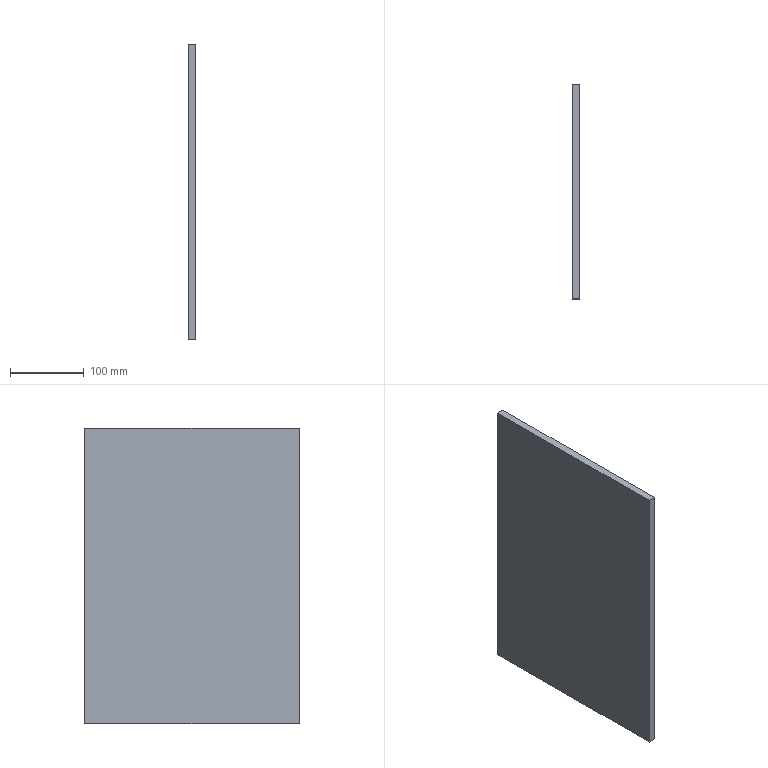Component | SolidWorks | BlockingPlate-5 | 1 solid | 6 faces | box 10 x 290 x 400 mm | volume 1160000 mm3 | plane 6 | material Plain Carbon Steel
STEP:
#1=COLOUR_RGB('',0.7922,0.8196,0.9333);
#2=FILL_AREA_STYLE_COLOUR('',#1);
#3=FILL_AREA_STYLE('',(#2));
#4=SURFACE_STYLE_FILL_AREA(#3);
#5=SURFACE_SIDE_STYLE('',(#4));
#6=SURFACE_STYLE_USAGE(.BOTH.,#5);
#7=PRESENTATION_STYLE_ASSIGNMENT((#6));
#8=CARTESIAN_POINT('',(671.454,114.953,65.169));
#9=VERTEX_POINT('',#8);
#10=CARTESIAN_POINT('',(671.454,126.37,65.169));
#11=VERTEX_POINT('',#10);
#12=CARTESIAN_POINT('',(671.454,126.37,65.169));
#13=DIRECTION('',(0.,1.,0.));
#14=VECTOR('',#13,39.37);
#15=LINE('',#12,#14);
#16=EDGE_CURVE('',#9,#11,#15,.T.);
#17=ORIENTED_EDGE('',*,*,#16,.F.);
#18=CARTESIAN_POINT('',(671.061,114.953,65.169));
#19=VERTEX_POINT('',#18);
#20=CARTESIAN_POINT('',(671.061,114.953,65.169));
#21=DIRECTION('',(1.,-0.,-0.));
#22=VECTOR('',#21,39.37);
#23=LINE('',#20,#22);
#24=EDGE_CURVE('',#19,#9,#23,.T.);
#25=ORIENTED_EDGE('',*,*,#24,.F.);
#26=CARTESIAN_POINT('',(671.061,126.37,65.169));
#27=VERTEX_POINT('',#26);
#28=CARTESIAN_POINT('',(671.061,126.37,65.169));
#29=DIRECTION('',(0.,1.,0.));
#30=VECTOR('',#29,39.37);
#31=LINE('',#28,#30);
#32=EDGE_CURVE('',#19,#27,#31,.T.);
#33=ORIENTED_EDGE('',*,*,#32,.T.);
#34=CARTESIAN_POINT('',(671.061,126.37,65.169));
#35=DIRECTION('',(1.,-0.,-0.));
#36=VECTOR('',#35,39.37);
#37=LINE('',#34,#36);
#38=EDGE_CURVE('',#27,#11,#37,.T.);
#39=ORIENTED_EDGE('',*,*,#38,.T.);
#40=EDGE_LOOP('',(#17,#25,#33,#39));
#41=FACE_OUTER_BOUND('',#40,.T.);
#42=CARTESIAN_POINT('',(671.061,126.37,65.169));
#43=DIRECTION('',(-0.,0.,-1.));
#44=DIRECTION('',(0.,1.,0.));
#45=AXIS2_PLACEMENT_3D('',#42,#43,#44);
#46=PLANE('',#45);
#47=ADVANCED_FACE('',(#41),#46,.T.);
#48=CARTESIAN_POINT('',(671.454,114.953,80.917));
#49=VERTEX_POINT('',#48);
#50=CARTESIAN_POINT('',(671.454,114.953,80.917));
#51=DIRECTION('',(-0.,0.,-1.));
#52=VECTOR('',#51,39.37);
#53=LINE('',#50,#52);
#54=EDGE_CURVE('',#49,#9,#53,.T.);
#55=ORIENTED_EDGE('',*,*,#54,.F.);
#56=CARTESIAN_POINT('',(671.061,114.953,80.917));
#57=VERTEX_POINT('',#56);
#58=CARTESIAN_POINT('',(671.061,114.953,80.917));
#59=DIRECTION('',(1.,-0.,-0.));
#60=VECTOR('',#59,39.37);
#61=LINE('',#58,#60);
#62=EDGE_CURVE('',#57,#49,#61,.T.);
#63=ORIENTED_EDGE('',*,*,#62,.F.);
#64=CARTESIAN_POINT('',(671.061,114.953,80.917));
#65=DIRECTION('',(-0.,0.,-1.));
#66=VECTOR('',#65,39.37);
#67=LINE('',#64,#66);
#68=EDGE_CURVE('',#57,#19,#67,.T.);
#69=ORIENTED_EDGE('',*,*,#68,.T.);
#70=ORIENTED_EDGE('',*,*,#24,.T.);
#71=EDGE_LOOP('',(#55,#63,#69,#70));
#72=FACE_OUTER_BOUND('',#71,.T.);
#73=CARTESIAN_POINT('',(671.061,114.953,80.917));
#74=DIRECTION('',(-0.,-1.,0.));
#75=DIRECTION('',(-0.,0.,-1.));
#76=AXIS2_PLACEMENT_3D('',#73,#74,#75);
#77=PLANE('',#76);
#78=ADVANCED_FACE('',(#72),#77,.T.);
#79=CARTESIAN_POINT('',(671.454,126.37,80.917));
#80=VERTEX_POINT('',#79);
#81=CARTESIAN_POINT('',(671.454,126.37,80.917));
#82=DIRECTION('',(-0.,-1.,-0.));
#83=VECTOR('',#82,39.37);
#84=LINE('',#81,#83);
#85=EDGE_CURVE('',#80,#49,#84,.T.);
#86=ORIENTED_EDGE('',*,*,#85,.F.);
#87=CARTESIAN_POINT('',(671.061,126.37,80.917));
#88=VERTEX_POINT('',#87);
#89=CARTESIAN_POINT('',(671.061,126.37,80.917));
#90=DIRECTION('',(1.,-0.,-0.));
#91=VECTOR('',#90,39.37);
#92=LINE('',#89,#91);
#93=EDGE_CURVE('',#88,#80,#92,.T.);
#94=ORIENTED_EDGE('',*,*,#93,.F.);
#95=CARTESIAN_POINT('',(671.061,126.37,80.917));
#96=DIRECTION('',(-0.,-1.,-0.));
#97=VECTOR('',#96,39.37);
#98=LINE('',#95,#97);
#99=EDGE_CURVE('',#88,#57,#98,.T.);
#100=ORIENTED_EDGE('',*,*,#99,.T.);
#101=ORIENTED_EDGE('',*,*,#62,.T.);
#102=EDGE_LOOP('',(#86,#94,#100,#101));
#103=FACE_OUTER_BOUND('',#102,.T.);
#104=CARTESIAN_POINT('',(671.061,126.37,80.917));
#105=DIRECTION('',(0.,-0.,1.));
#106=DIRECTION('',(-0.,-1.,-0.));
#107=AXIS2_PLACEMENT_3D('',#104,#105,#106);
#108=PLANE('',#107);
#109=ADVANCED_FACE('',(#103),#108,.T.);
#110=CARTESIAN_POINT('',(671.454,126.37,80.917));
#111=DIRECTION('',(0.,0.,1.));
#112=VECTOR('',#111,39.37);
#113=LINE('',#110,#112);
#114=EDGE_CURVE('',#11,#80,#113,.T.);
#115=ORIENTED_EDGE('',*,*,#114,.F.);
#116=ORIENTED_EDGE('',*,*,#38,.F.);
#117=CARTESIAN_POINT('',(671.061,126.37,80.917));
#118=DIRECTION('',(0.,0.,1.));
#119=VECTOR('',#118,39.37);
#120=LINE('',#117,#119);
#121=EDGE_CURVE('',#27,#88,#120,.T.);
#122=ORIENTED_EDGE('',*,*,#121,.T.);
#123=ORIENTED_EDGE('',*,*,#93,.T.);
#124=EDGE_LOOP('',(#115,#116,#122,#123));
#125=FACE_OUTER_BOUND('',#124,.T.);
#126=CARTESIAN_POINT('',(671.061,126.37,80.917));
#127=DIRECTION('',(0.,1.,-0.));
#128=DIRECTION('',(0.,0.,1.));
#129=AXIS2_PLACEMENT_3D('',#126,#127,#128);
#130=PLANE('',#129);
#131=ADVANCED_FACE('',(#125),#130,.T.);
#132=ORIENTED_EDGE('',*,*,#32,.F.);
#133=ORIENTED_EDGE('',*,*,#68,.F.);
#134=ORIENTED_EDGE('',*,*,#99,.F.);
#135=ORIENTED_EDGE('',*,*,#121,.F.);
#136=EDGE_LOOP('',(#132,#133,#134,#135));
#137=FACE_OUTER_BOUND('',#136,.T.);
#138=CARTESIAN_POINT('',(671.061,120.662,73.043));
#139=DIRECTION('',(1.,-0.,-0.));
#140=DIRECTION('',(-0.,-1.,0.));
#141=AXIS2_PLACEMENT_3D('',#138,#139,#140);
#142=PLANE('',#141);
#143=ADVANCED_FACE('',(#137),#142,.F.);
#144=ORIENTED_EDGE('',*,*,#16,.T.);
#145=ORIENTED_EDGE('',*,*,#114,.T.);
#146=ORIENTED_EDGE('',*,*,#85,.T.);
#147=ORIENTED_EDGE('',*,*,#54,.T.);
#148=EDGE_LOOP('',(#144,#145,#146,#147));
#149=FACE_OUTER_BOUND('',#148,.T.);
#150=CARTESIAN_POINT('',(671.454,120.662,73.043));
#151=DIRECTION('',(1.,-0.,-0.));
#152=DIRECTION('',(-0.,-1.,0.));
#153=AXIS2_PLACEMENT_3D('',#150,#151,#152);
#154=PLANE('',#153);
#155=ADVANCED_FACE('',(#149),#154,.T.);
#156=CLOSED_SHELL('',(#47,#78,#109,#131,#143,#155));
#157=MANIFOLD_SOLID_BREP('',#156);
#158=STYLED_ITEM('',(#7),#157);
#159=(LENGTH_UNIT()NAMED_UNIT(*)SI_UNIT($,.METRE.));
#160=LENGTH_MEASURE_WITH_UNIT(LENGTH_MEASURE(0.0254),#159);
#161=DIMENSIONAL_EXPONENTS(1.,0.,0.,0.,0.,0.,0.);
#162=(CONVERSION_BASED_UNIT('',#160)LENGTH_UNIT()NAMED_UNIT(#161));
#163=UNCERTAINTY_MEASURE_WITH_UNIT(LENGTH_MEASURE(0.00001),#162,'','');
#164=(NAMED_UNIT(*)PLANE_ANGLE_UNIT()SI_UNIT($,.RADIAN.));
#165=(NAMED_UNIT(*)SI_UNIT($,.STERADIAN.)SOLID_ANGLE_UNIT());
#166=(GEOMETRIC_REPRESENTATION_CONTEXT(3)GLOBAL_UNCERTAINTY_ASSIGNED_CONTEXT((#163))GLOBAL_UNIT_ASSIGNED_CONTEXT((#162,#164,#165))REPRESENTATION_CONTEXT('',''));
#167=MECHANICAL_DESIGN_GEOMETRIC_PRESENTATION_REPRESENTATION('',(#158),#166);
#168=PRESENTATION_LAYER_ASSIGNMENT('','',(#158));
#169=CARTESIAN_POINT('',(0.,0.,0.));
#170=DIRECTION('',(0.,0.,1.));
#171=DIRECTION('',(1.,0.,0.));
#172=AXIS2_PLACEMENT_3D('',#169,#170,#171);
#173=(LENGTH_UNIT()NAMED_UNIT(*)SI_UNIT($,.METRE.));
#174=LENGTH_MEASURE_WITH_UNIT(LENGTH_MEASURE(0.0254),#173);
#175=DIMENSIONAL_EXPONENTS(1.,0.,0.,0.,0.,0.,0.);
#176=(CONVERSION_BASED_UNIT('',#174)LENGTH_UNIT()NAMED_UNIT(#175));
#177=UNCERTAINTY_MEASURE_WITH_UNIT(LENGTH_MEASURE(0.00001),#176,'','');
#178=(NAMED_UNIT(*)PLANE_ANGLE_UNIT()SI_UNIT($,.RADIAN.));
#179=(NAMED_UNIT(*)SI_UNIT($,.STERADIAN.)SOLID_ANGLE_UNIT());
#180=(GEOMETRIC_REPRESENTATION_CONTEXT(3)GLOBAL_UNCERTAINTY_ASSIGNED_CONTEXT((#177))GLOBAL_UNIT_ASSIGNED_CONTEXT((#176,#178,#179))REPRESENTATION_CONTEXT('',''));
#181=ADVANCED_BREP_SHAPE_REPRESENTATION('',(#157,#172),#180);